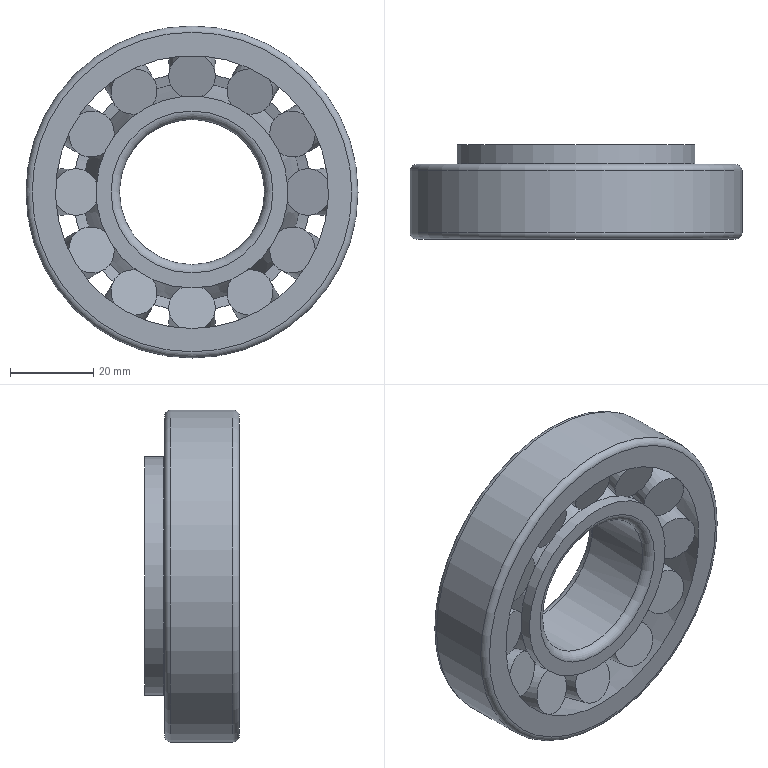Component | NX | BEARING_30307_2 | 14 solids | 52 faces | volume 58197 mm3 | plane 28 | cylinder 16 | cone 4 | torus 4 | commonest cylinder face diameters 11.25 x12 80 x1 57.5 x1 46.25 x1 35 x1